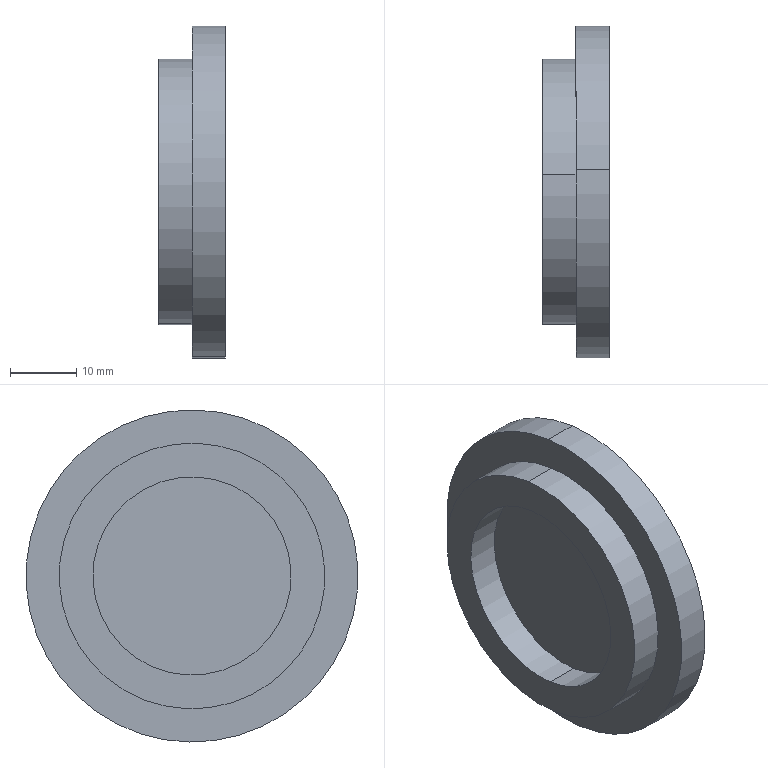Component | SolidWorks | EndCover-1 | 1 solid | 10 faces | box 10 x 50 x 50 mm | volume 12604 mm3 | cylinder 6 | plane 4 | commonest cylinder face diameters 29.84 x2 50 x2 40 x2
build123d program:
from build123d import *

# Parameters (mm, degrees)
SKETCH1_R               = 20
BOSS_EXTRUDE1_DEPTH     = 5
SKETCH2_R               = 25
BOSS_EXTRUDE2_DEPTH     = 5
CUT_EXTRUDE1_DEPTH      = 37.742
CUT_EXTRUDE1_DEPTH_BACK = 5
SKETCH3_R               = 14.92


with BuildPart() as part:
    # Sketch1 → Boss-Extrude1 (new body)
    with BuildSketch(Plane.XY):
        Circle(SKETCH1_R)
    extrude(amount=BOSS_EXTRUDE1_DEPTH)

    # Sketch2 → Boss-Extrude2 (add)
    with BuildSketch(Plane.XY.offset(5)):
        Circle(SKETCH2_R)
    extrude(amount=BOSS_EXTRUDE2_DEPTH)

    # Sketch3 → Cut-Extrude1 (cut, two sides: drawn at the far end of the back side and taken through both)
    with BuildSketch(Plane(origin=(0, 0, 0), x_dir=(-1, 0, 0), z_dir=(0, 0, -1)).offset(-CUT_EXTRUDE1_DEPTH_BACK)):
        with Locations(Location((0, 0, 0), (0, 0, 180))):
            Circle(SKETCH3_R)
    extrude(amount=CUT_EXTRUDE1_DEPTH + CUT_EXTRUDE1_DEPTH_BACK, mode=Mode.SUBTRACT)


solid = part.part

# Placed as in the assembly
solid = solid.moved(Location((529.39, 335.1, -35), (0, 90, 0)))
STEP:
#1=COLOUR_RGB('',0.7922,0.8196,0.9333);
#2=FILL_AREA_STYLE_COLOUR('',#1);
#3=FILL_AREA_STYLE('',(#2));
#4=SURFACE_STYLE_FILL_AREA(#3);
#5=SURFACE_SIDE_STYLE('',(#4));
#6=SURFACE_STYLE_USAGE(.BOTH.,#5);
#7=PRESENTATION_STYLE_ASSIGNMENT((#6));
#8=CARTESIAN_POINT('',(20.842,13.271,-0.7958));
#9=VERTEX_POINT('',#8);
#10=CARTESIAN_POINT('',(20.842,13.115,-1.96));
#11=VERTEX_POINT('',#10);
#12=CARTESIAN_POINT('',(20.842,13.193,-1.378));
#13=DIRECTION('',(-1.,-0.,-0.));
#14=DIRECTION('',(0.,0.1334,0.9911));
#15=AXIS2_PLACEMENT_3D('',#12,#13,#14);
#16=CIRCLE('',#15,0.5874);
#17=EDGE_CURVE('',#9,#11,#16,.T.);
#18=ORIENTED_EDGE('',*,*,#17,.T.);
#19=CARTESIAN_POINT('',(21.039,13.115,-1.96));
#20=VERTEX_POINT('',#19);
#21=CARTESIAN_POINT('',(20.842,13.115,-1.96));
#22=DIRECTION('',(1.,0.,0.));
#23=VECTOR('',#22,39.37);
#24=LINE('',#21,#23);
#25=EDGE_CURVE('',#11,#20,#24,.T.);
#26=ORIENTED_EDGE('',*,*,#25,.T.);
#27=CARTESIAN_POINT('',(21.039,13.271,-0.7958));
#28=VERTEX_POINT('',#27);
#29=CARTESIAN_POINT('',(21.039,13.193,-1.378));
#30=DIRECTION('',(-1.,-0.,-0.));
#31=DIRECTION('',(0.,-0.1334,-0.9911));
#32=AXIS2_PLACEMENT_3D('',#29,#30,#31);
#33=CIRCLE('',#32,0.5874);
#34=EDGE_CURVE('',#28,#20,#33,.T.);
#35=ORIENTED_EDGE('',*,*,#34,.F.);
#36=CARTESIAN_POINT('',(20.842,13.271,-0.7958));
#37=DIRECTION('',(1.,0.,0.));
#38=VECTOR('',#37,39.37);
#39=LINE('',#36,#38);
#40=EDGE_CURVE('',#9,#28,#39,.T.);
#41=ORIENTED_EDGE('',*,*,#40,.F.);
#42=EDGE_LOOP('',(#18,#26,#35,#41));
#43=FACE_OUTER_BOUND('',#42,.T.);
#44=CARTESIAN_POINT('',(20.842,13.193,-1.378));
#45=DIRECTION('',(1.,0.,0.));
#46=DIRECTION('',(0.,0.1334,0.9911));
#47=AXIS2_PLACEMENT_3D('',#44,#45,#46);
#48=CYLINDRICAL_SURFACE('',#47,0.5874);
#49=ADVANCED_FACE('',(#43),#48,.F.);
#50=CARTESIAN_POINT('',(21.236,13.324,-0.4025));
#51=VERTEX_POINT('',#50);
#52=CARTESIAN_POINT('',(21.236,13.062,-2.353));
#53=VERTEX_POINT('',#52);
#54=CARTESIAN_POINT('',(21.236,13.193,-1.378));
#55=DIRECTION('',(1.,0.,0.));
#56=DIRECTION('',(0.,0.1334,0.9911));
#57=AXIS2_PLACEMENT_3D('',#54,#55,#56);
#58=CIRCLE('',#57,0.9843);
#59=EDGE_CURVE('',#51,#53,#58,.T.);
#60=ORIENTED_EDGE('',*,*,#59,.F.);
#61=CARTESIAN_POINT('',(21.039,13.324,-0.4025));
#62=VERTEX_POINT('',#61);
#63=CARTESIAN_POINT('',(21.236,13.324,-0.4025));
#64=DIRECTION('',(-1.,-0.,-0.));
#65=VECTOR('',#64,39.37);
#66=LINE('',#63,#65);
#67=EDGE_CURVE('',#51,#62,#66,.T.);
#68=ORIENTED_EDGE('',*,*,#67,.T.);
#69=CARTESIAN_POINT('',(21.039,13.062,-2.353));
#70=VERTEX_POINT('',#69);
#71=CARTESIAN_POINT('',(21.039,13.193,-1.378));
#72=DIRECTION('',(1.,0.,0.));
#73=DIRECTION('',(0.,0.1334,0.9911));
#74=AXIS2_PLACEMENT_3D('',#71,#72,#73);
#75=CIRCLE('',#74,0.9843);
#76=EDGE_CURVE('',#62,#70,#75,.T.);
#77=ORIENTED_EDGE('',*,*,#76,.T.);
#78=CARTESIAN_POINT('',(21.236,13.062,-2.353));
#79=DIRECTION('',(-1.,-0.,-0.));
#80=VECTOR('',#79,39.37);
#81=LINE('',#78,#80);
#82=EDGE_CURVE('',#53,#70,#81,.T.);
#83=ORIENTED_EDGE('',*,*,#82,.F.);
#84=EDGE_LOOP('',(#60,#68,#77,#83));
#85=FACE_OUTER_BOUND('',#84,.T.);
#86=CARTESIAN_POINT('',(21.236,13.193,-1.378));
#87=DIRECTION('',(-1.,-0.,-0.));
#88=DIRECTION('',(0.,-0.1334,-0.9911));
#89=AXIS2_PLACEMENT_3D('',#86,#87,#88);
#90=CYLINDRICAL_SURFACE('',#89,0.9843);
#91=ADVANCED_FACE('',(#85),#90,.T.);
#92=CARTESIAN_POINT('',(21.039,13.298,-0.5976));
#93=VERTEX_POINT('',#92);
#94=CARTESIAN_POINT('',(21.039,13.088,-2.158));
#95=VERTEX_POINT('',#94);
#96=CARTESIAN_POINT('',(21.039,13.193,-1.378));
#97=DIRECTION('',(1.,0.,0.));
#98=DIRECTION('',(0.,0.1334,0.9911));
#99=AXIS2_PLACEMENT_3D('',#96,#97,#98);
#100=CIRCLE('',#99,0.7874);
#101=EDGE_CURVE('',#93,#95,#100,.T.);
#102=ORIENTED_EDGE('',*,*,#101,.F.);
#103=CARTESIAN_POINT('',(20.842,13.298,-0.5976));
#104=VERTEX_POINT('',#103);
#105=CARTESIAN_POINT('',(21.039,13.298,-0.5976));
#106=DIRECTION('',(-1.,-0.,-0.));
#107=VECTOR('',#106,39.37);
#108=LINE('',#105,#107);
#109=EDGE_CURVE('',#93,#104,#108,.T.);
#110=ORIENTED_EDGE('',*,*,#109,.T.);
#111=CARTESIAN_POINT('',(20.842,13.088,-2.158));
#112=VERTEX_POINT('',#111);
#113=CARTESIAN_POINT('',(20.842,13.193,-1.378));
#114=DIRECTION('',(1.,0.,0.));
#115=DIRECTION('',(0.,0.1334,0.9911));
#116=AXIS2_PLACEMENT_3D('',#113,#114,#115);
#117=CIRCLE('',#116,0.7874);
#118=EDGE_CURVE('',#104,#112,#117,.T.);
#119=ORIENTED_EDGE('',*,*,#118,.T.);
#120=CARTESIAN_POINT('',(21.039,13.088,-2.158));
#121=DIRECTION('',(-1.,-0.,-0.));
#122=VECTOR('',#121,39.37);
#123=LINE('',#120,#122);
#124=EDGE_CURVE('',#95,#112,#123,.T.);
#125=ORIENTED_EDGE('',*,*,#124,.F.);
#126=EDGE_LOOP('',(#102,#110,#119,#125));
#127=FACE_OUTER_BOUND('',#126,.T.);
#128=CARTESIAN_POINT('',(21.039,13.193,-1.378));
#129=DIRECTION('',(-1.,-0.,-0.));
#130=DIRECTION('',(0.,-0.1334,-0.9911));
#131=AXIS2_PLACEMENT_3D('',#128,#129,#130);
#132=CYLINDRICAL_SURFACE('',#131,0.7874);
#133=ADVANCED_FACE('',(#127),#132,.T.);
#134=ORIENTED_EDGE('',*,*,#109,.F.);
#135=CARTESIAN_POINT('',(21.039,13.193,-1.378));
#136=DIRECTION('',(1.,0.,0.));
#137=DIRECTION('',(0.,0.1334,0.9911));
#138=AXIS2_PLACEMENT_3D('',#135,#136,#137);
#139=CIRCLE('',#138,0.7874);
#140=EDGE_CURVE('',#95,#93,#139,.T.);
#141=ORIENTED_EDGE('',*,*,#140,.F.);
#142=ORIENTED_EDGE('',*,*,#124,.T.);
#143=CARTESIAN_POINT('',(20.842,13.193,-1.378));
#144=DIRECTION('',(1.,0.,0.));
#145=DIRECTION('',(0.,0.1334,0.9911));
#146=AXIS2_PLACEMENT_3D('',#143,#144,#145);
#147=CIRCLE('',#146,0.7874);
#148=EDGE_CURVE('',#112,#104,#147,.T.);
#149=ORIENTED_EDGE('',*,*,#148,.T.);
#150=EDGE_LOOP('',(#134,#141,#142,#149));
#151=FACE_OUTER_BOUND('',#150,.T.);
#152=CARTESIAN_POINT('',(21.039,13.193,-1.378));
#153=DIRECTION('',(-1.,-0.,-0.));
#154=DIRECTION('',(0.,-0.1334,-0.9911));
#155=AXIS2_PLACEMENT_3D('',#152,#153,#154);
#156=CYLINDRICAL_SURFACE('',#155,0.7874);
#157=ADVANCED_FACE('',(#151),#156,.T.);
#158=ORIENTED_EDGE('',*,*,#17,.F.);
#159=CARTESIAN_POINT('',(20.842,13.193,-1.378));
#160=DIRECTION('',(-1.,-0.,-0.));
#161=DIRECTION('',(0.,0.1334,0.9911));
#162=AXIS2_PLACEMENT_3D('',#159,#160,#161);
#163=CIRCLE('',#162,0.5874);
#164=EDGE_CURVE('',#11,#9,#163,.T.);
#165=ORIENTED_EDGE('',*,*,#164,.F.);
#166=EDGE_LOOP('',(#158,#165));
#167=FACE_BOUND('',#166,.T.);
#168=ORIENTED_EDGE('',*,*,#148,.F.);
#169=ORIENTED_EDGE('',*,*,#118,.F.);
#170=EDGE_LOOP('',(#168,#169));
#171=FACE_OUTER_BOUND('',#170,.T.);
#172=CARTESIAN_POINT('',(20.842,13.193,-1.378));
#173=DIRECTION('',(1.,0.,0.));
#174=DIRECTION('',(-0.,0.1334,0.9911));
#175=AXIS2_PLACEMENT_3D('',#172,#173,#174);
#176=PLANE('',#175);
#177=ADVANCED_FACE('',(#167,#171),#176,.F.);
#178=ORIENTED_EDGE('',*,*,#67,.F.);
#179=CARTESIAN_POINT('',(21.236,13.193,-1.378));
#180=DIRECTION('',(1.,0.,0.));
#181=DIRECTION('',(0.,0.1334,0.9911));
#182=AXIS2_PLACEMENT_3D('',#179,#180,#181);
#183=CIRCLE('',#182,0.9843);
#184=EDGE_CURVE('',#53,#51,#183,.T.);
#185=ORIENTED_EDGE('',*,*,#184,.F.);
#186=ORIENTED_EDGE('',*,*,#82,.T.);
#187=CARTESIAN_POINT('',(21.039,13.193,-1.378));
#188=DIRECTION('',(1.,0.,0.));
#189=DIRECTION('',(0.,0.1334,0.9911));
#190=AXIS2_PLACEMENT_3D('',#187,#188,#189);
#191=CIRCLE('',#190,0.9843);
#192=EDGE_CURVE('',#70,#62,#191,.T.);
#193=ORIENTED_EDGE('',*,*,#192,.T.);
#194=EDGE_LOOP('',(#178,#185,#186,#193));
#195=FACE_OUTER_BOUND('',#194,.T.);
#196=CARTESIAN_POINT('',(21.236,13.193,-1.378));
#197=DIRECTION('',(-1.,-0.,-0.));
#198=DIRECTION('',(0.,-0.1334,-0.9911));
#199=AXIS2_PLACEMENT_3D('',#196,#197,#198);
#200=CYLINDRICAL_SURFACE('',#199,0.9843);
#201=ADVANCED_FACE('',(#195),#200,.T.);
#202=ORIENTED_EDGE('',*,*,#184,.T.);
#203=ORIENTED_EDGE('',*,*,#59,.T.);
#204=EDGE_LOOP('',(#202,#203));
#205=FACE_OUTER_BOUND('',#204,.T.);
#206=CARTESIAN_POINT('',(21.236,13.193,-1.378));
#207=DIRECTION('',(1.,0.,0.));
#208=DIRECTION('',(-0.,0.1334,0.9911));
#209=AXIS2_PLACEMENT_3D('',#206,#207,#208);
#210=PLANE('',#209);
#211=ADVANCED_FACE('',(#205),#210,.T.);
#212=ORIENTED_EDGE('',*,*,#140,.T.);
#213=ORIENTED_EDGE('',*,*,#101,.T.);
#214=EDGE_LOOP('',(#212,#213));
#215=FACE_BOUND('',#214,.T.);
#216=ORIENTED_EDGE('',*,*,#192,.F.);
#217=ORIENTED_EDGE('',*,*,#76,.F.);
#218=EDGE_LOOP('',(#216,#217));
#219=FACE_OUTER_BOUND('',#218,.T.);
#220=CARTESIAN_POINT('',(21.039,13.193,-1.378));
#221=DIRECTION('',(1.,0.,0.));
#222=DIRECTION('',(-0.,0.1334,0.9911));
#223=AXIS2_PLACEMENT_3D('',#220,#221,#222);
#224=PLANE('',#223);
#225=ADVANCED_FACE('',(#215,#219),#224,.F.);
#226=ORIENTED_EDGE('',*,*,#25,.F.);
#227=ORIENTED_EDGE('',*,*,#164,.T.);
#228=ORIENTED_EDGE('',*,*,#40,.T.);
#229=CARTESIAN_POINT('',(21.039,13.193,-1.378));
#230=DIRECTION('',(-1.,-0.,-0.));
#231=DIRECTION('',(0.,-0.1334,-0.9911));
#232=AXIS2_PLACEMENT_3D('',#229,#230,#231);
#233=CIRCLE('',#232,0.5874);
#234=EDGE_CURVE('',#20,#28,#233,.T.);
#235=ORIENTED_EDGE('',*,*,#234,.F.);
#236=EDGE_LOOP('',(#226,#227,#228,#235));
#237=FACE_OUTER_BOUND('',#236,.T.);
#238=CARTESIAN_POINT('',(20.842,13.193,-1.378));
#239=DIRECTION('',(1.,0.,0.));
#240=DIRECTION('',(0.,0.1334,0.9911));
#241=AXIS2_PLACEMENT_3D('',#238,#239,#240);
#242=CYLINDRICAL_SURFACE('',#241,0.5874);
#243=ADVANCED_FACE('',(#237),#242,.F.);
#244=ORIENTED_EDGE('',*,*,#34,.T.);
#245=ORIENTED_EDGE('',*,*,#234,.T.);
#246=EDGE_LOOP('',(#244,#245));
#247=FACE_OUTER_BOUND('',#246,.T.);
#248=CARTESIAN_POINT('',(21.039,13.193,-1.378));
#249=DIRECTION('',(-1.,-0.,-0.));
#250=DIRECTION('',(0.,-0.1334,-0.9911));
#251=AXIS2_PLACEMENT_3D('',#248,#249,#250);
#252=PLANE('',#251);
#253=ADVANCED_FACE('',(#247),#252,.T.);
#254=CLOSED_SHELL('',(#49,#91,#133,#157,#177,#201,#211,#225,#243,#253));
#255=MANIFOLD_SOLID_BREP('',#254);
#256=STYLED_ITEM('',(#7),#255);
#257=PRESENTATION_LAYER_ASSIGNMENT('','',(#256));
#258=(LENGTH_UNIT()NAMED_UNIT(*)SI_UNIT($,.METRE.));
#259=LENGTH_MEASURE_WITH_UNIT(LENGTH_MEASURE(0.0254),#258);
#260=DIMENSIONAL_EXPONENTS(1.,0.,0.,0.,0.,0.,0.);
#261=(CONVERSION_BASED_UNIT('',#259)LENGTH_UNIT()NAMED_UNIT(#260));
#262=UNCERTAINTY_MEASURE_WITH_UNIT(LENGTH_MEASURE(0.00001),#261,'','');
#263=(NAMED_UNIT(*)PLANE_ANGLE_UNIT()SI_UNIT($,.RADIAN.));
#264=(NAMED_UNIT(*)SI_UNIT($,.STERADIAN.)SOLID_ANGLE_UNIT());
#265=(GEOMETRIC_REPRESENTATION_CONTEXT(3)GLOBAL_UNCERTAINTY_ASSIGNED_CONTEXT((#262))GLOBAL_UNIT_ASSIGNED_CONTEXT((#261,#263,#264))REPRESENTATION_CONTEXT('',''));
#266=MECHANICAL_DESIGN_GEOMETRIC_PRESENTATION_REPRESENTATION('',(#256),#265);
#267=CARTESIAN_POINT('',(0.,0.,0.));
#268=DIRECTION('',(0.,0.,1.));
#269=DIRECTION('',(1.,0.,0.));
#270=AXIS2_PLACEMENT_3D('',#267,#268,#269);
#271=(LENGTH_UNIT()NAMED_UNIT(*)SI_UNIT($,.METRE.));
#272=LENGTH_MEASURE_WITH_UNIT(LENGTH_MEASURE(0.0254),#271);
#273=DIMENSIONAL_EXPONENTS(1.,0.,0.,0.,0.,0.,0.);
#274=(CONVERSION_BASED_UNIT('',#272)LENGTH_UNIT()NAMED_UNIT(#273));
#275=UNCERTAINTY_MEASURE_WITH_UNIT(LENGTH_MEASURE(0.00001),#274,'','');
#276=(NAMED_UNIT(*)PLANE_ANGLE_UNIT()SI_UNIT($,.RADIAN.));
#277=(NAMED_UNIT(*)SI_UNIT($,.STERADIAN.)SOLID_ANGLE_UNIT());
#278=(GEOMETRIC_REPRESENTATION_CONTEXT(3)GLOBAL_UNCERTAINTY_ASSIGNED_CONTEXT((#275))GLOBAL_UNIT_ASSIGNED_CONTEXT((#274,#276,#277))REPRESENTATION_CONTEXT('',''));
#279=ADVANCED_BREP_SHAPE_REPRESENTATION('',(#255,#270),#278);